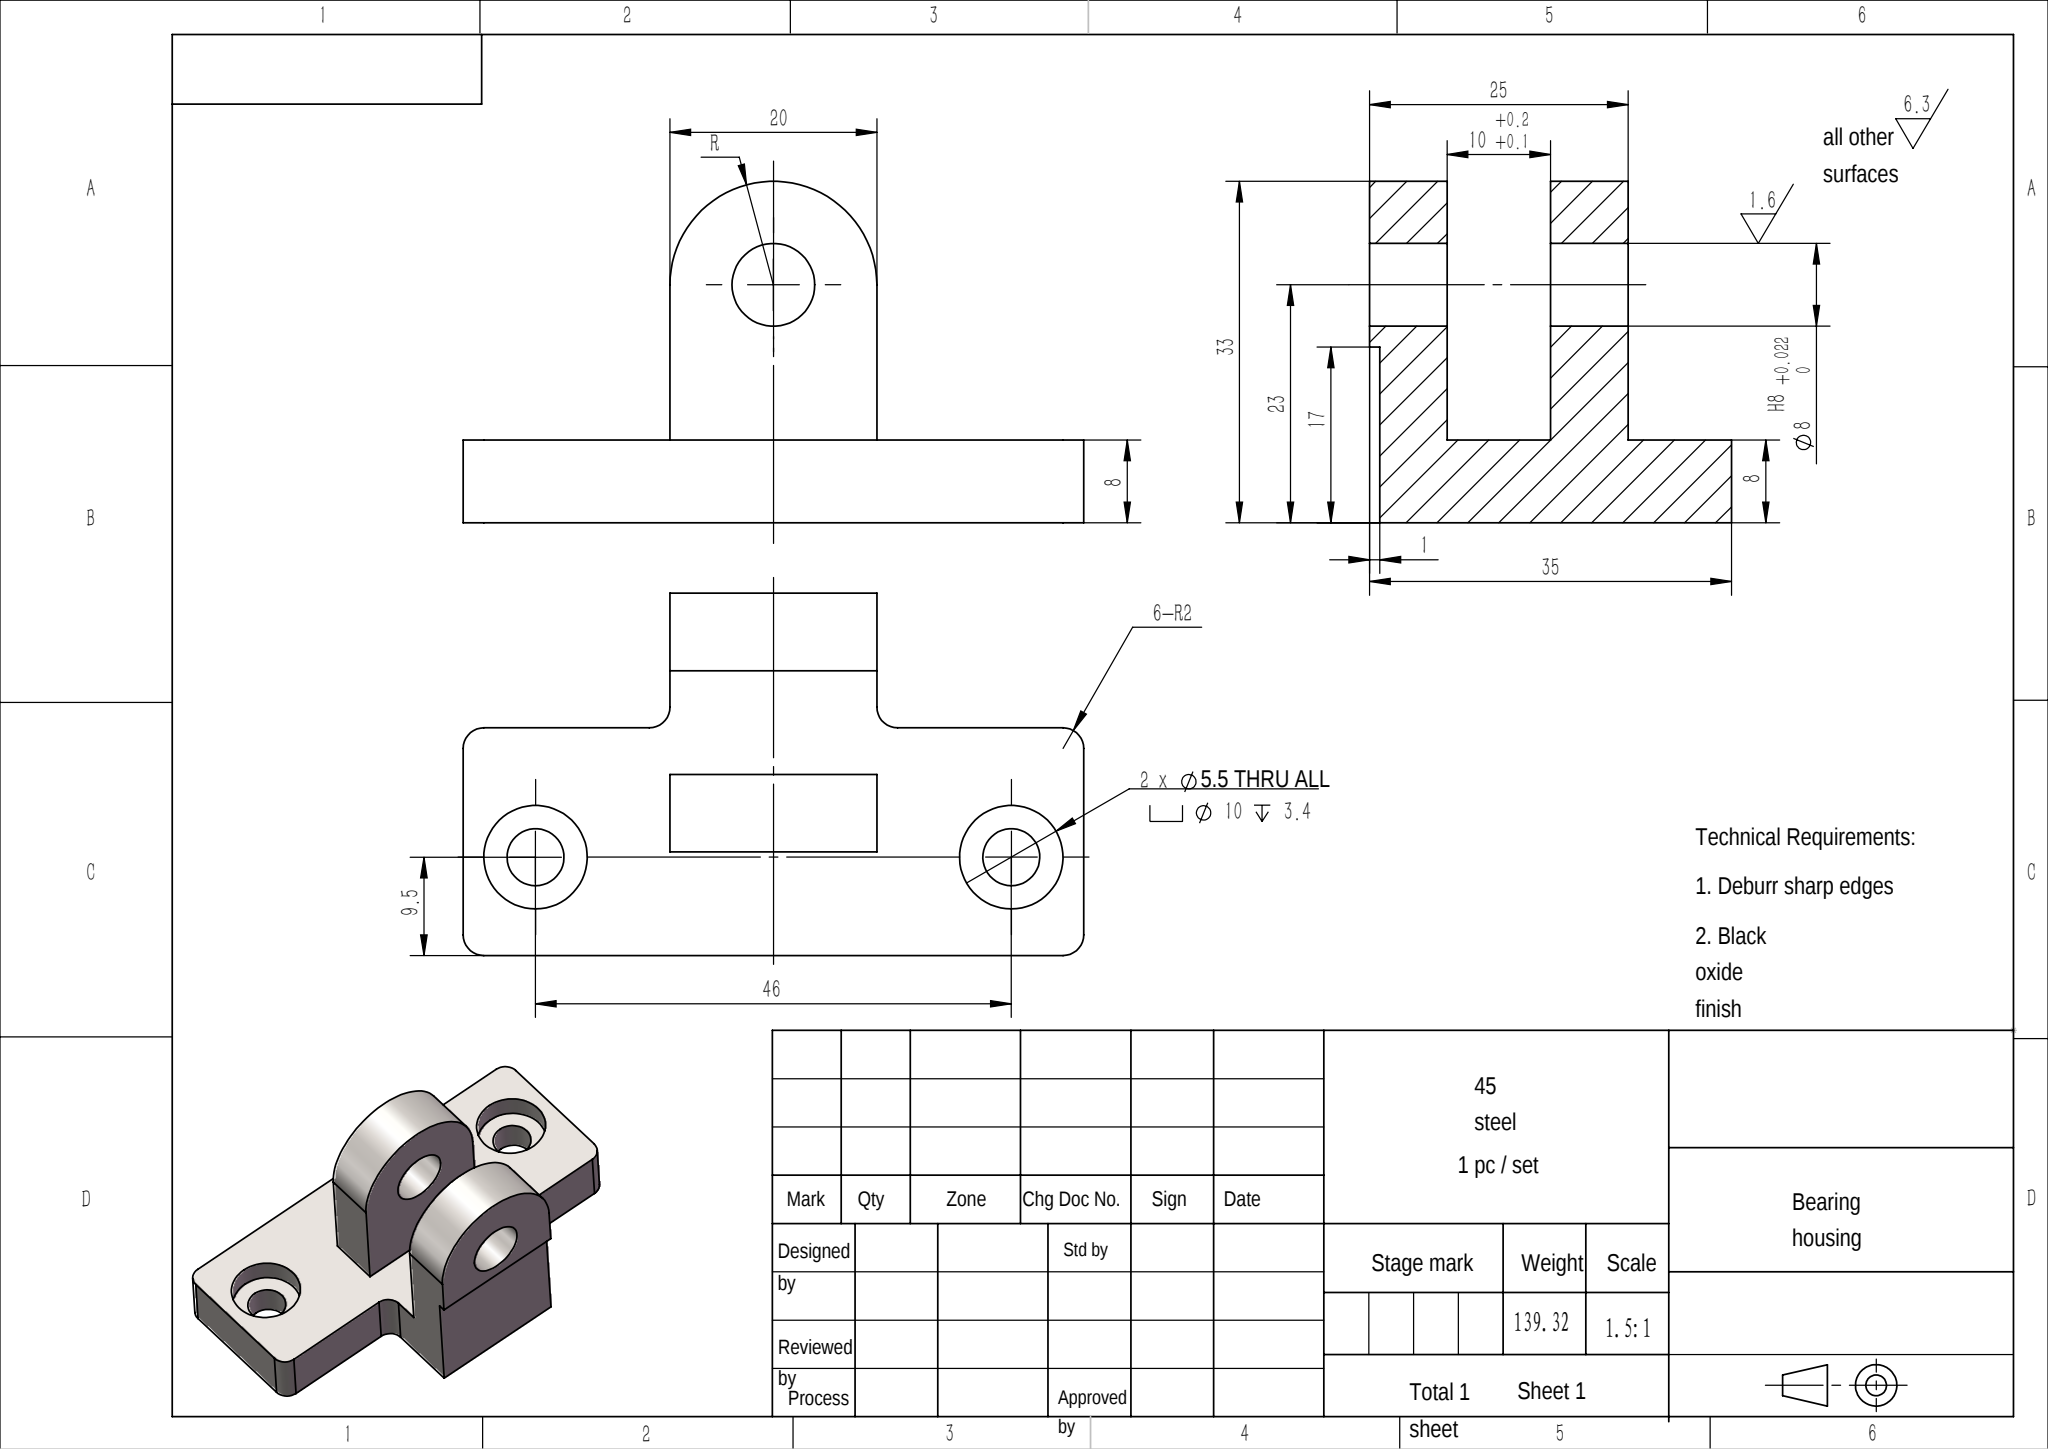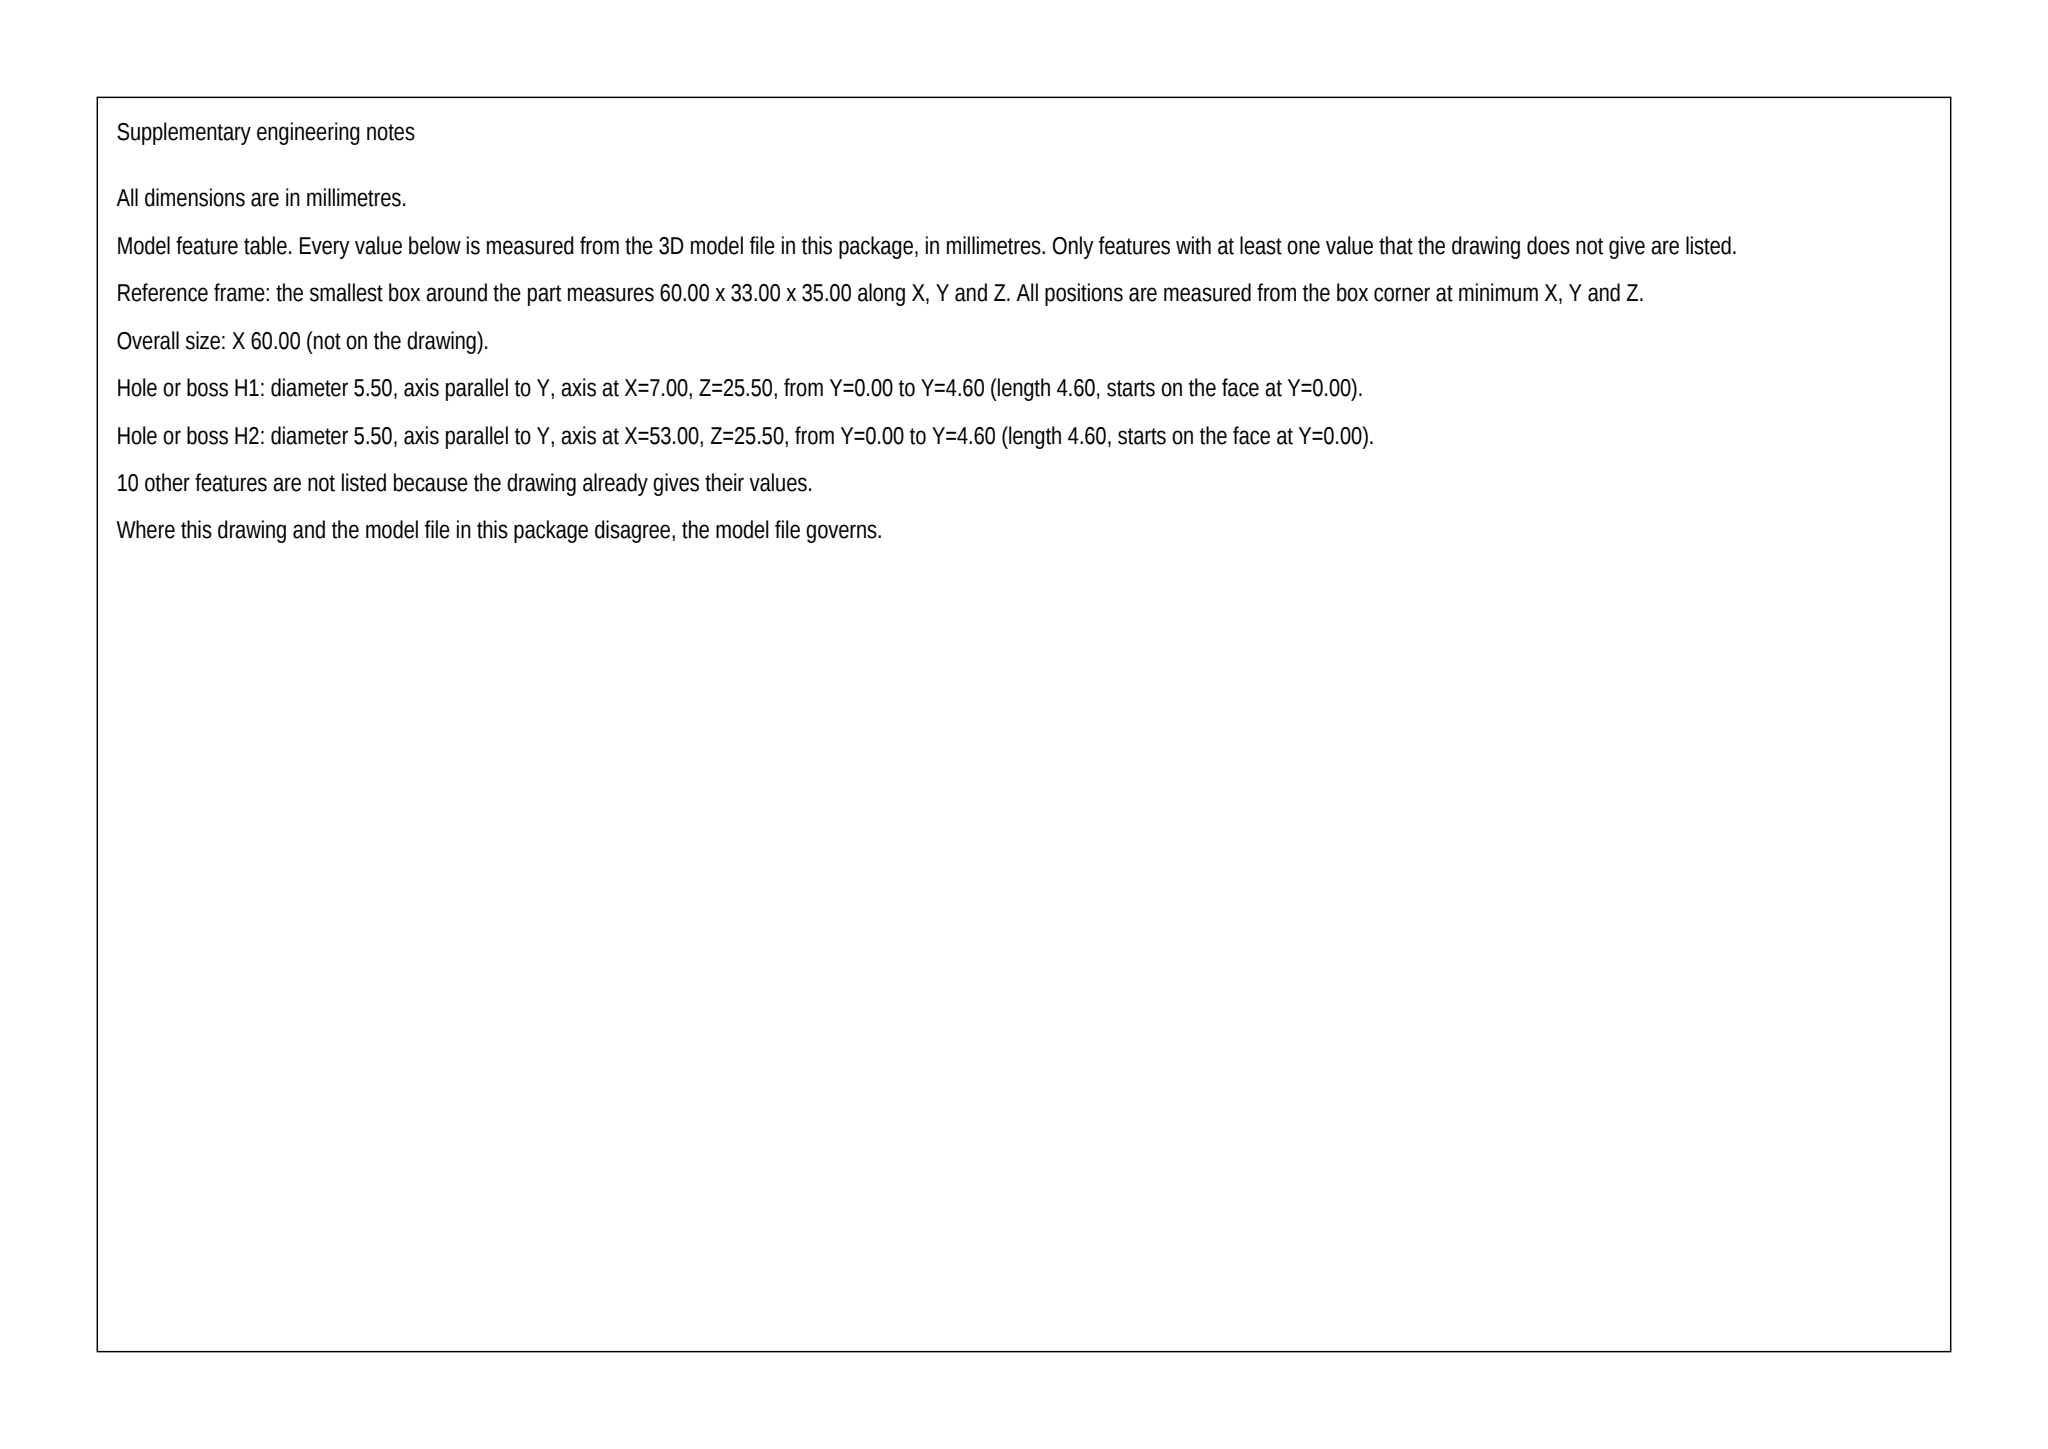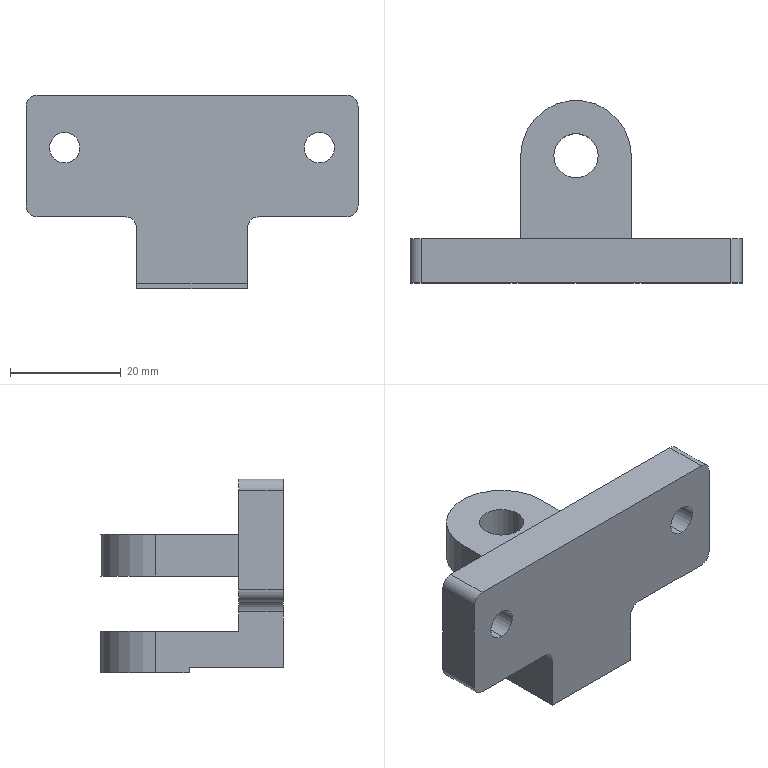Part | SolidWorks | mm | material 45 steel | 1 solid | 39 faces | box 60 x 33 x 35 mm | volume 17636 mm3 | cylinder 20 | plane 19 | commonest cylinder face diameters 4 x6 10 x4 5.5 x4 8 x4 20 x2
build123d program:
from build123d import *

# Parameters (mm, degrees)
BOSS_EXTRUDE1_DEPTH                             = 12.5
SKETCH2_W                                       = 20
SKETCH2_H                                       = 60
CUT_EXTRUDE1_DEPTH                              = 5
F_8_0_8_DIAMETER_HOLE1_D                        = 8
SKETCH5_W                                       = 60
SKETCH5_H                                       = 25
BOSS_EXTRUDE2_DEPTH                             = 8
SKETCH8_W                                       = 60
SKETCH8_H                                       = 10
BOSS_EXTRUDE3_DEPTH                             = 8
M5_HEX_SOCKET_HEAD_CAP_SCREW_CBORE1_D           = 5.5
M5_HEX_SOCKET_HEAD_CAP_SCREW_CBORE1_CBORE_D     = 10
M5_HEX_SOCKET_HEAD_CAP_SCREW_CBORE1_CBORE_DEPTH = 3.4
SKETCH9_W                                       = 20
SKETCH9_H                                       = 13
CUT_EXTRUDE2_DEPTH                              = 46.069
FILLET2_R                                       = 2
FILLET3_R                                       = 2
SKETCH10_W                                      = 20
SKETCH10_H                                      = 17
CUT_EXTRUDE3_DEPTH                              = 1


with BuildPart() as part:
    # Sketch1 → Boss-Extrude1 (new, symmetric)
    with BuildSketch(Plane.XY):
        with BuildLine():
            Line((-10, 0), (10, 0))
            Line((10, 0), (10, 23))
            ThreePointArc((10, 23), (0, 33), (-10, 23))
            Line((-10, 23), (-10, 0))
        make_face()
    extrude(amount=BOSS_EXTRUDE1_DEPTH, both=True)

    # Sketch2 → Cut-Extrude1 (cut, symmetric)
    with BuildSketch(Plane.XY):
        with Locations((0, 38)):
            Rectangle(SKETCH2_W, SKETCH2_H)
    extrude(amount=CUT_EXTRUDE1_DEPTH, both=True, mode=Mode.SUBTRACT)

    # 8.0 _8_ Diameter Hole1 (through all)
    with Locations(Plane.XY.offset(12.5)):
        with Locations((0, 23)):
            Hole(F_8_0_8_DIAMETER_HOLE1_D / 2)

    # Sketch5 → Boss-Extrude2 (add)
    with BuildSketch(Plane.XZ):
        Rectangle(SKETCH5_W, SKETCH5_H)
    extrude(amount=-BOSS_EXTRUDE2_DEPTH)

    # Sketch8 → Boss-Extrude3 (add)
    with BuildSketch(Plane(origin=(0, 8, 0), x_dir=(1, 0, 0), z_dir=(0, 1, 0))):
        with Locations((0, -17.5)):
            Rectangle(SKETCH8_W, SKETCH8_H)
    extrude(amount=-BOSS_EXTRUDE3_DEPTH)

    # M5 Hex Socket Head Cap Screw CBORE1 (through all)
    with Locations(Plane(origin=(0, 8, 0), x_dir=(1, 0, 0), z_dir=(0, 1, 0))):
        with Locations((23, -13), (-23, -13)):
            CounterBoreHole(M5_HEX_SOCKET_HEAD_CAP_SCREW_CBORE1_D / 2, M5_HEX_SOCKET_HEAD_CAP_SCREW_CBORE1_CBORE_D / 2, M5_HEX_SOCKET_HEAD_CAP_SCREW_CBORE1_CBORE_DEPTH)

    # Sketch9 → Cut-Extrude2 (cut, through all)
    with BuildSketch(Plane(origin=(0, 8, 0), x_dir=(1, 0, 0), z_dir=(0, 1, 0))):
        with Locations((20, 6)):
            Rectangle(SKETCH9_W, SKETCH9_H)
        with Locations((-20, 6)):
            Rectangle(SKETCH9_W, SKETCH9_H)
    extrude(amount=-CUT_EXTRUDE2_DEPTH, mode=Mode.SUBTRACT)

    # Fillet2
    fillet2_edges = [part.edges().sort_by_distance(p)[0] for p in [
        (10, 4, 0.5),
        (-10, 4, 0.5),
    ]]
    fillet(fillet2_edges, radius=FILLET2_R)

    # Fillet3
    fillet3_edges = [part.edges().sort_by_distance(p)[0] for p in [
        (30, 4, 0.5),
        (-30, 4, 0.5),
        (-30, 4, 22.5),
        (30, 4, 22.5),
    ]]
    fillet(fillet3_edges, radius=FILLET3_R)

    # Sketch10 → Cut-Extrude3 (cut)
    with BuildSketch(Plane(origin=(0, 0, -12.5), x_dir=(-1, 0, 0), z_dir=(0, 0, -1))):
        with Locations((0, 8.5)):
            Rectangle(SKETCH10_W, SKETCH10_H)
    extrude(amount=-CUT_EXTRUDE3_DEPTH, mode=Mode.SUBTRACT)


solid = part.part